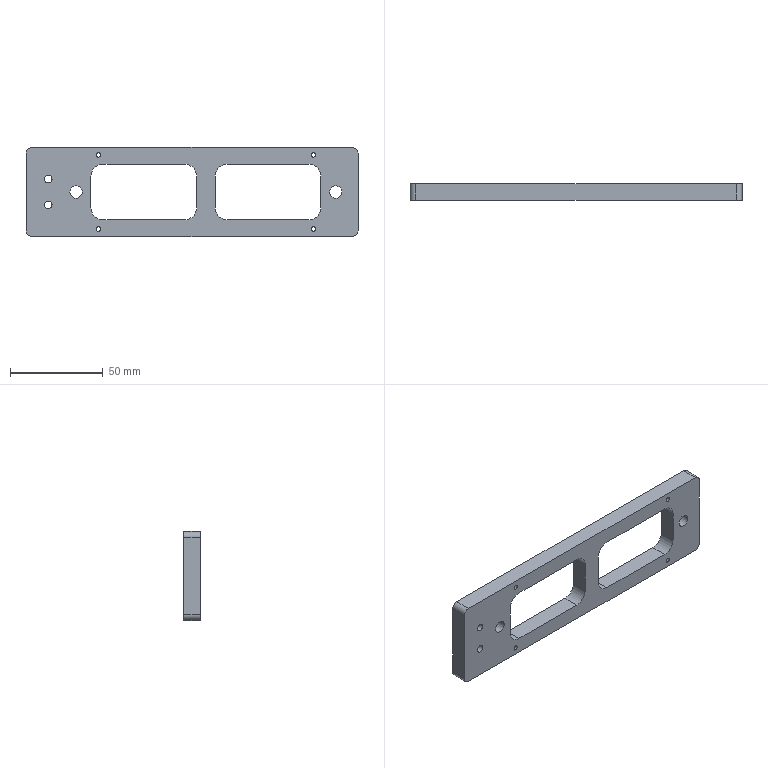CAM job | Mastercam | mm | 8 operations | part box 179 x 9 x 48
1. Facing | 24 - 100 平铣刀
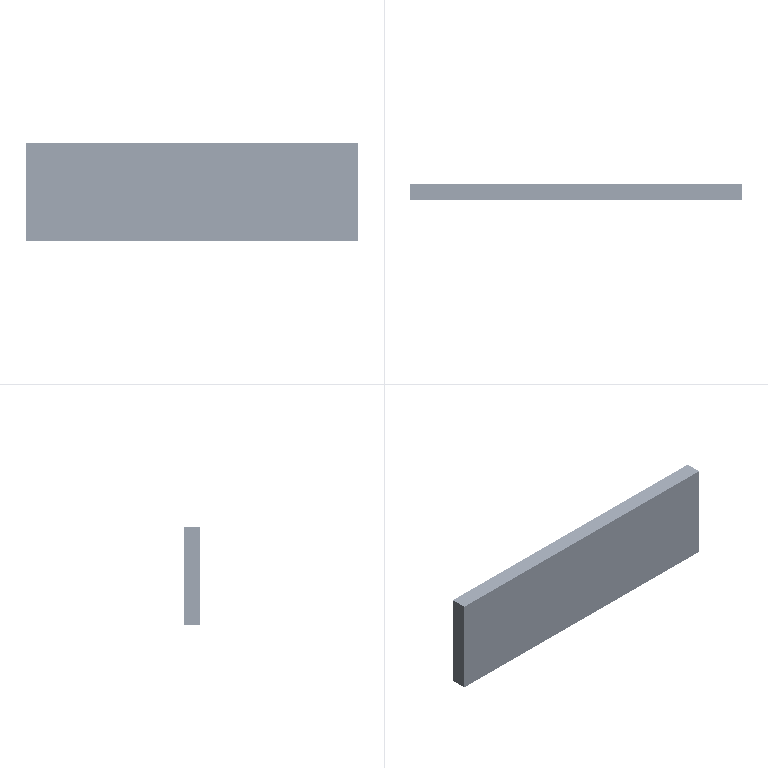2. Contour (Ramp) | 12 - 12 平铣刀
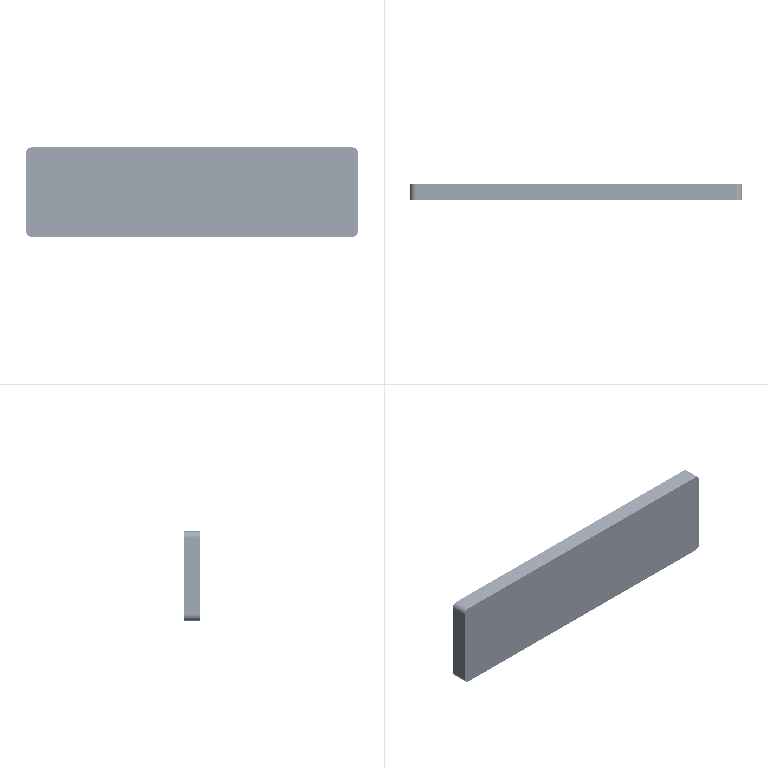3. 2D High Speed (2D Dynamic Mill) | 12 - 12 平铣刀
4. Contour (2D) | 10 - 10 平铣刀
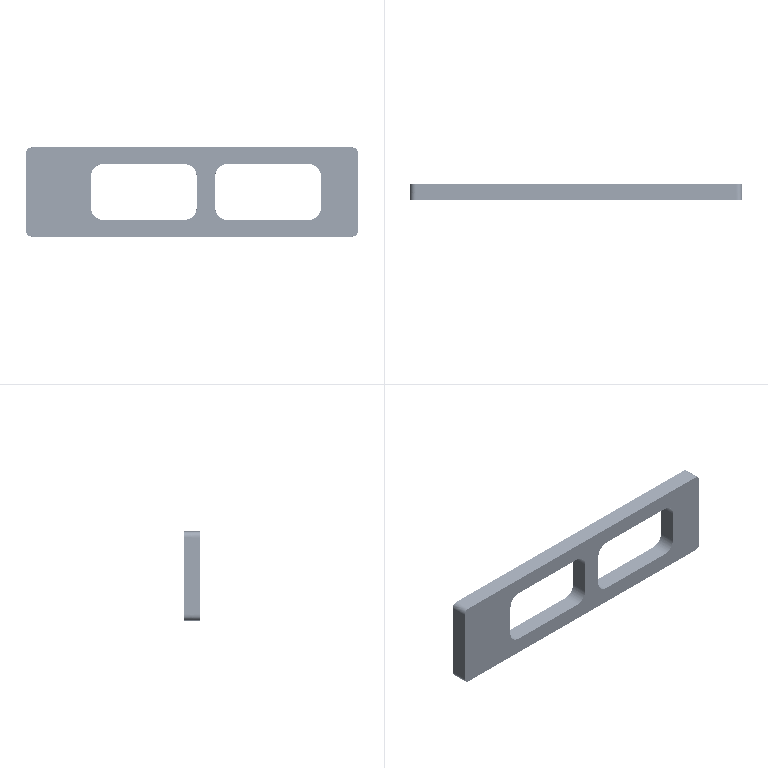5. Drill/Counterbore | 7 - 4 倒角刀
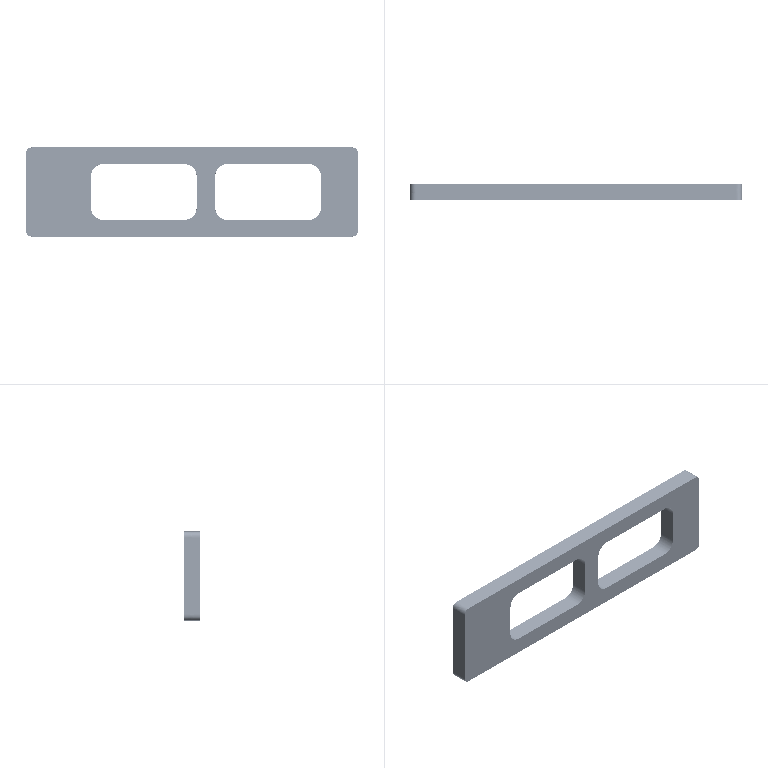6. Contour (2D chamfer) | 7 - 4 倒角刀
7. Facing | 24 - 100 平铣刀
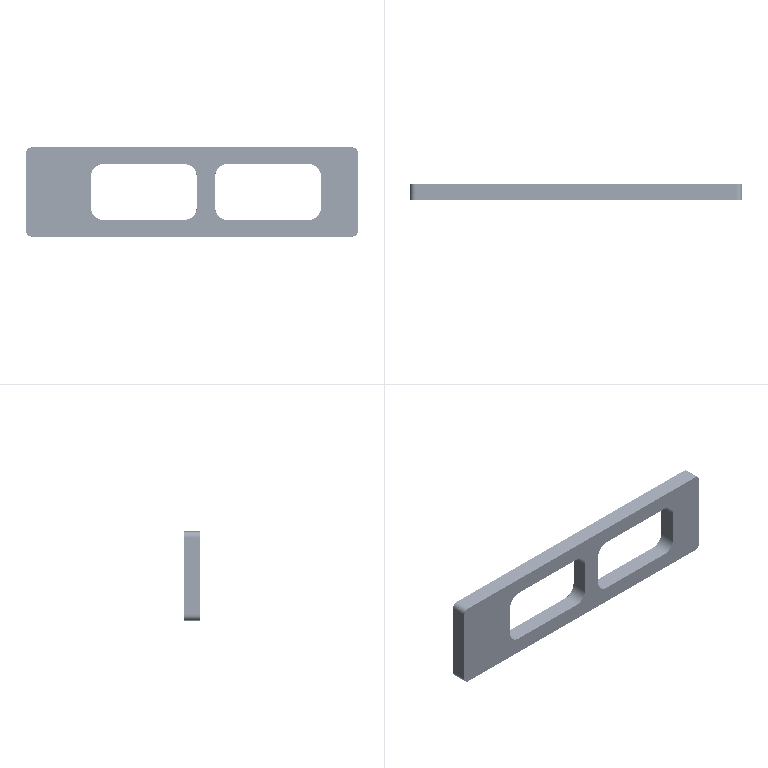8. Contour (2D chamfer) | 7 - 4 倒角刀